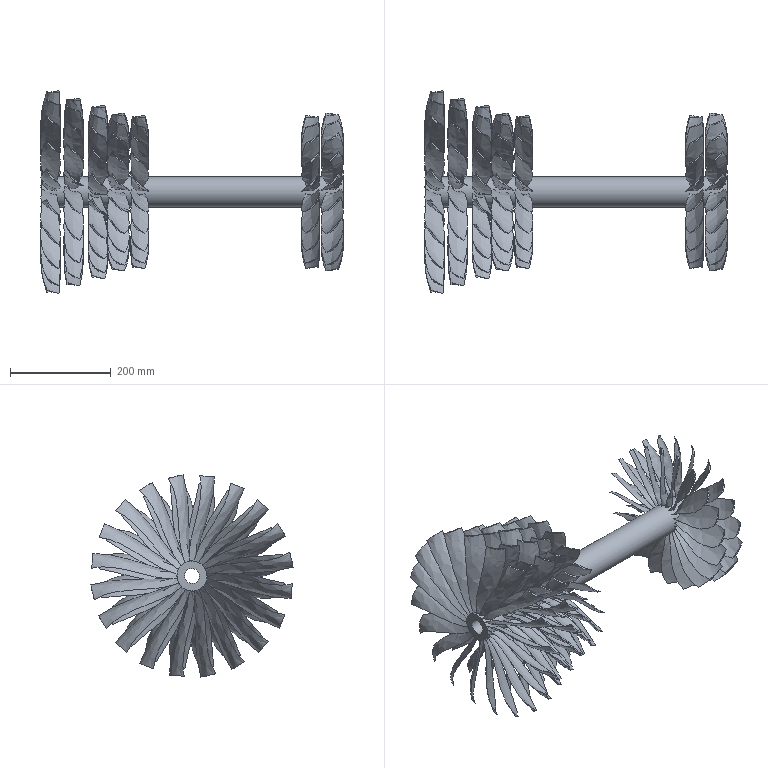Component | NX | COMP_AND_TURB | 1 solid | 427 faces | volume 2614419 mm3 | spline 280 | plane 142 | cylinder 5 | commonest cylinder face diameters 60 x4 30 x1